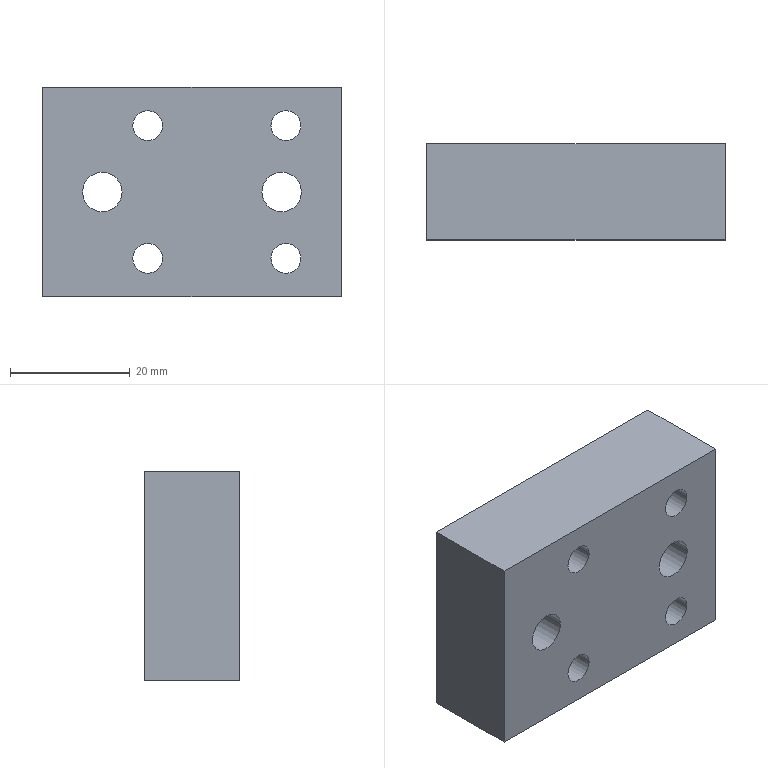Component | SolidWorks | QuickClampBackingPlate-1 | 1 solid | 24 faces | box 50 x 16 x 35 mm | volume 24821 mm3 | cylinder 16 | plane 8 | commonest cylinder face diameters 5 x8 11 x4 6.6 x4 | material 6061 Alloy
build123d program:
from build123d import *

# Parameters (mm, degrees)
SKETCH1_W                                          = 50
SKETCH1_H                                          = 35
BOSS_EXTRUDE1_DEPTH                                = 8
HOLE_SIZE_ACCORDING_TO_TYPE_1_OF_HEXAG_D           = 6.6
HOLE_SIZE_ACCORDING_TO_TYPE_1_OF_HEXAG_DEPTH       = 20
HOLE_SIZE_ACCORDING_TO_TYPE_1_OF_HEXAG_CBORE_D     = 11
HOLE_SIZE_ACCORDING_TO_TYPE_1_OF_HEXAG_CBORE_DEPTH = 6.8
HOLE_SIZE_ACCORDING_TO_TYPE_1_OF_HEXAG_TIP         = 1.983
M6_TAPPED_HOLE1_D                                  = 5
M6_TAPPED_HOLE1_DEPTH                              = 21
M6_TAPPED_HOLE1_TIP                                = 1.502


with BuildPart() as part:
    # Sketch1 → Boss-Extrude1 (new, symmetric)
    with BuildSketch(Plane.XY):
        Rectangle(SKETCH1_W, SKETCH1_H)
    extrude(amount=BOSS_EXTRUDE1_DEPTH, both=True)

    # Hole Size _according to_ Type 1 of Hexag
    with Locations(Plane(origin=(0, 0, -8), x_dir=(1, 0, 0), z_dir=(0, 0, -1))):
        with Locations((-15, 0), (15, 0)):
            CounterBoreHole(HOLE_SIZE_ACCORDING_TO_TYPE_1_OF_HEXAG_D / 2, HOLE_SIZE_ACCORDING_TO_TYPE_1_OF_HEXAG_CBORE_D / 2, HOLE_SIZE_ACCORDING_TO_TYPE_1_OF_HEXAG_CBORE_DEPTH, depth=HOLE_SIZE_ACCORDING_TO_TYPE_1_OF_HEXAG_DEPTH)
            with Locations((0, 0, -(HOLE_SIZE_ACCORDING_TO_TYPE_1_OF_HEXAG_DEPTH + HOLE_SIZE_ACCORDING_TO_TYPE_1_OF_HEXAG_TIP / 2))):  # 118° drill point
                Cone(0, HOLE_SIZE_ACCORDING_TO_TYPE_1_OF_HEXAG_D / 2, HOLE_SIZE_ACCORDING_TO_TYPE_1_OF_HEXAG_TIP, mode=Mode.SUBTRACT)

    # M6 Tapped Hole1
    with Locations(Plane(origin=(0, 0, -8), x_dir=(-1, 0, 0), z_dir=(0, 0, -1))):
        with Locations((-15.7, 11.1), (7.4, 11.1), (-15.7, -11.1), (7.4, -11.1)):
            Hole(M6_TAPPED_HOLE1_D / 2, depth=M6_TAPPED_HOLE1_DEPTH)
            with Locations((0, 0, -(M6_TAPPED_HOLE1_DEPTH + M6_TAPPED_HOLE1_TIP / 2))):  # 118° drill point
                Cone(0, M6_TAPPED_HOLE1_D / 2, M6_TAPPED_HOLE1_TIP, mode=Mode.SUBTRACT)


solid = part.part

# Placed as in the assembly
solid = solid.moved(Location((36.028, 36.101, 117.932), (90, 0, 0)))
STEP:
#1=COLOUR_RGB('',0.7922,0.8196,0.9333);
#2=FILL_AREA_STYLE_COLOUR('',#1);
#3=FILL_AREA_STYLE('',(#2));
#4=SURFACE_STYLE_FILL_AREA(#3);
#5=SURFACE_SIDE_STYLE('',(#4));
#6=SURFACE_STYLE_USAGE(.BOTH.,#5);
#7=PRESENTATION_STYLE_ASSIGNMENT((#6));
#8=CARTESIAN_POINT('',(2.135,1.106,5.08));
#9=VERTEX_POINT('',#8);
#10=CARTESIAN_POINT('',(1.938,1.106,5.08));
#11=VERTEX_POINT('',#10);
#12=CARTESIAN_POINT('',(2.037,1.106,5.08));
#13=DIRECTION('',(0.,1.,0.));
#14=DIRECTION('',(-1.,0.,0.));
#15=AXIS2_PLACEMENT_3D('',#12,#13,#14);
#16=CIRCLE('',#15,0.09843);
#17=EDGE_CURVE('',#9,#11,#16,.T.);
#18=ORIENTED_EDGE('',*,*,#17,.F.);
#19=CARTESIAN_POINT('',(2.135,1.736,5.08));
#20=VERTEX_POINT('',#19);
#21=CARTESIAN_POINT('',(2.135,1.736,5.08));
#22=DIRECTION('',(0.,1.,0.));
#23=VECTOR('',#22,39.37);
#24=LINE('',#21,#23);
#25=EDGE_CURVE('',#9,#20,#24,.T.);
#26=ORIENTED_EDGE('',*,*,#25,.T.);
#27=CARTESIAN_POINT('',(1.938,1.736,5.08));
#28=VERTEX_POINT('',#27);
#29=CARTESIAN_POINT('',(2.037,1.736,5.08));
#30=DIRECTION('',(0.,1.,0.));
#31=DIRECTION('',(-1.,0.,0.));
#32=AXIS2_PLACEMENT_3D('',#29,#30,#31);
#33=CIRCLE('',#32,0.09843);
#34=EDGE_CURVE('',#20,#28,#33,.T.);
#35=ORIENTED_EDGE('',*,*,#34,.T.);
#36=CARTESIAN_POINT('',(1.938,1.736,5.08));
#37=DIRECTION('',(0.,1.,0.));
#38=VECTOR('',#37,39.37);
#39=LINE('',#36,#38);
#40=EDGE_CURVE('',#11,#28,#39,.T.);
#41=ORIENTED_EDGE('',*,*,#40,.F.);
#42=EDGE_LOOP('',(#18,#26,#35,#41));
#43=FACE_OUTER_BOUND('',#42,.T.);
#44=CARTESIAN_POINT('',(2.037,1.736,5.08));
#45=DIRECTION('',(0.,1.,0.));
#46=DIRECTION('',(-1.,0.,0.));
#47=AXIS2_PLACEMENT_3D('',#44,#45,#46);
#48=CYLINDRICAL_SURFACE('',#47,0.09843);
#49=ADVANCED_FACE('',(#43),#48,.F.);
#50=CARTESIAN_POINT('',(1.226,1.106,5.08));
#51=VERTEX_POINT('',#50);
#52=CARTESIAN_POINT('',(1.029,1.106,5.08));
#53=VERTEX_POINT('',#52);
#54=CARTESIAN_POINT('',(1.127,1.106,5.08));
#55=DIRECTION('',(0.,1.,0.));
#56=DIRECTION('',(-1.,0.,0.));
#57=AXIS2_PLACEMENT_3D('',#54,#55,#56);
#58=CIRCLE('',#57,0.09843);
#59=EDGE_CURVE('',#51,#53,#58,.T.);
#60=ORIENTED_EDGE('',*,*,#59,.F.);
#61=CARTESIAN_POINT('',(1.226,1.736,5.08));
#62=VERTEX_POINT('',#61);
#63=CARTESIAN_POINT('',(1.226,1.736,5.08));
#64=DIRECTION('',(0.,1.,0.));
#65=VECTOR('',#64,39.37);
#66=LINE('',#63,#65);
#67=EDGE_CURVE('',#51,#62,#66,.T.);
#68=ORIENTED_EDGE('',*,*,#67,.T.);
#69=CARTESIAN_POINT('',(1.029,1.736,5.08));
#70=VERTEX_POINT('',#69);
#71=CARTESIAN_POINT('',(1.127,1.736,5.08));
#72=DIRECTION('',(0.,1.,0.));
#73=DIRECTION('',(-1.,0.,0.));
#74=AXIS2_PLACEMENT_3D('',#71,#72,#73);
#75=CIRCLE('',#74,0.09843);
#76=EDGE_CURVE('',#62,#70,#75,.T.);
#77=ORIENTED_EDGE('',*,*,#76,.T.);
#78=CARTESIAN_POINT('',(1.029,1.736,5.08));
#79=DIRECTION('',(0.,1.,0.));
#80=VECTOR('',#79,39.37);
#81=LINE('',#78,#80);
#82=EDGE_CURVE('',#53,#70,#81,.T.);
#83=ORIENTED_EDGE('',*,*,#82,.F.);
#84=EDGE_LOOP('',(#60,#68,#77,#83));
#85=FACE_OUTER_BOUND('',#84,.T.);
#86=CARTESIAN_POINT('',(1.127,1.736,5.08));
#87=DIRECTION('',(0.,1.,0.));
#88=DIRECTION('',(-1.,0.,0.));
#89=AXIS2_PLACEMENT_3D('',#86,#87,#88);
#90=CYLINDRICAL_SURFACE('',#89,0.09843);
#91=ADVANCED_FACE('',(#85),#90,.F.);
#92=CARTESIAN_POINT('',(2.135,1.106,4.206));
#93=VERTEX_POINT('',#92);
#94=CARTESIAN_POINT('',(1.938,1.106,4.206));
#95=VERTEX_POINT('',#94);
#96=CARTESIAN_POINT('',(2.037,1.106,4.206));
#97=DIRECTION('',(0.,1.,0.));
#98=DIRECTION('',(-1.,0.,0.));
#99=AXIS2_PLACEMENT_3D('',#96,#97,#98);
#100=CIRCLE('',#99,0.09843);
#101=EDGE_CURVE('',#93,#95,#100,.T.);
#102=ORIENTED_EDGE('',*,*,#101,.F.);
#103=CARTESIAN_POINT('',(2.135,1.736,4.206));
#104=VERTEX_POINT('',#103);
#105=CARTESIAN_POINT('',(2.135,1.736,4.206));
#106=DIRECTION('',(0.,1.,0.));
#107=VECTOR('',#106,39.37);
#108=LINE('',#105,#107);
#109=EDGE_CURVE('',#93,#104,#108,.T.);
#110=ORIENTED_EDGE('',*,*,#109,.T.);
#111=CARTESIAN_POINT('',(1.938,1.736,4.206));
#112=VERTEX_POINT('',#111);
#113=CARTESIAN_POINT('',(2.037,1.736,4.206));
#114=DIRECTION('',(0.,1.,0.));
#115=DIRECTION('',(-1.,0.,0.));
#116=AXIS2_PLACEMENT_3D('',#113,#114,#115);
#117=CIRCLE('',#116,0.09843);
#118=EDGE_CURVE('',#104,#112,#117,.T.);
#119=ORIENTED_EDGE('',*,*,#118,.T.);
#120=CARTESIAN_POINT('',(1.938,1.736,4.206));
#121=DIRECTION('',(0.,1.,0.));
#122=VECTOR('',#121,39.37);
#123=LINE('',#120,#122);
#124=EDGE_CURVE('',#95,#112,#123,.T.);
#125=ORIENTED_EDGE('',*,*,#124,.F.);
#126=EDGE_LOOP('',(#102,#110,#119,#125));
#127=FACE_OUTER_BOUND('',#126,.T.);
#128=CARTESIAN_POINT('',(2.037,1.736,4.206));
#129=DIRECTION('',(0.,1.,0.));
#130=DIRECTION('',(-1.,0.,0.));
#131=AXIS2_PLACEMENT_3D('',#128,#129,#130);
#132=CYLINDRICAL_SURFACE('',#131,0.09843);
#133=ADVANCED_FACE('',(#127),#132,.F.);
#134=CARTESIAN_POINT('',(1.226,1.106,4.206));
#135=VERTEX_POINT('',#134);
#136=CARTESIAN_POINT('',(1.029,1.106,4.206));
#137=VERTEX_POINT('',#136);
#138=CARTESIAN_POINT('',(1.127,1.106,4.206));
#139=DIRECTION('',(0.,1.,0.));
#140=DIRECTION('',(-1.,0.,0.));
#141=AXIS2_PLACEMENT_3D('',#138,#139,#140);
#142=CIRCLE('',#141,0.09843);
#143=EDGE_CURVE('',#135,#137,#142,.T.);
#144=ORIENTED_EDGE('',*,*,#143,.F.);
#145=CARTESIAN_POINT('',(1.226,1.736,4.206));
#146=VERTEX_POINT('',#145);
#147=CARTESIAN_POINT('',(1.226,1.736,4.206));
#148=DIRECTION('',(0.,1.,0.));
#149=VECTOR('',#148,39.37);
#150=LINE('',#147,#149);
#151=EDGE_CURVE('',#135,#146,#150,.T.);
#152=ORIENTED_EDGE('',*,*,#151,.T.);
#153=CARTESIAN_POINT('',(1.029,1.736,4.206));
#154=VERTEX_POINT('',#153);
#155=CARTESIAN_POINT('',(1.127,1.736,4.206));
#156=DIRECTION('',(0.,1.,0.));
#157=DIRECTION('',(-1.,0.,0.));
#158=AXIS2_PLACEMENT_3D('',#155,#156,#157);
#159=CIRCLE('',#158,0.09843);
#160=EDGE_CURVE('',#146,#154,#159,.T.);
#161=ORIENTED_EDGE('',*,*,#160,.T.);
#162=CARTESIAN_POINT('',(1.029,1.736,4.206));
#163=DIRECTION('',(0.,1.,0.));
#164=VECTOR('',#163,39.37);
#165=LINE('',#162,#164);
#166=EDGE_CURVE('',#137,#154,#165,.T.);
#167=ORIENTED_EDGE('',*,*,#166,.F.);
#168=EDGE_LOOP('',(#144,#152,#161,#167));
#169=FACE_OUTER_BOUND('',#168,.T.);
#170=CARTESIAN_POINT('',(1.127,1.736,4.206));
#171=DIRECTION('',(0.,1.,0.));
#172=DIRECTION('',(-1.,0.,0.));
#173=AXIS2_PLACEMENT_3D('',#170,#171,#172);
#174=CYLINDRICAL_SURFACE('',#173,0.09843);
#175=ADVANCED_FACE('',(#169),#174,.F.);
#176=CARTESIAN_POINT('',(1.044,1.469,4.643));
#177=VERTEX_POINT('',#176);
#178=CARTESIAN_POINT('',(0.6113,1.469,4.643));
#179=VERTEX_POINT('',#178);
#180=CARTESIAN_POINT('',(0.8279,1.469,4.643));
#181=DIRECTION('',(0.,1.,0.));
#182=DIRECTION('',(-1.,0.,0.));
#183=AXIS2_PLACEMENT_3D('',#180,#181,#182);
#184=CIRCLE('',#183,0.2165);
#185=EDGE_CURVE('',#177,#179,#184,.T.);
#186=ORIENTED_EDGE('',*,*,#185,.F.);
#187=CARTESIAN_POINT('',(1.044,1.736,4.643));
#188=VERTEX_POINT('',#187);
#189=CARTESIAN_POINT('',(1.044,1.736,4.643));
#190=DIRECTION('',(0.,1.,0.));
#191=VECTOR('',#190,39.37);
#192=LINE('',#189,#191);
#193=EDGE_CURVE('',#177,#188,#192,.T.);
#194=ORIENTED_EDGE('',*,*,#193,.T.);
#195=CARTESIAN_POINT('',(0.6113,1.736,4.643));
#196=VERTEX_POINT('',#195);
#197=CARTESIAN_POINT('',(0.8279,1.736,4.643));
#198=DIRECTION('',(0.,1.,0.));
#199=DIRECTION('',(-1.,0.,0.));
#200=AXIS2_PLACEMENT_3D('',#197,#198,#199);
#201=CIRCLE('',#200,0.2165);
#202=EDGE_CURVE('',#188,#196,#201,.T.);
#203=ORIENTED_EDGE('',*,*,#202,.T.);
#204=CARTESIAN_POINT('',(0.6113,1.736,4.643));
#205=DIRECTION('',(0.,1.,0.));
#206=VECTOR('',#205,39.37);
#207=LINE('',#204,#206);
#208=EDGE_CURVE('',#179,#196,#207,.T.);
#209=ORIENTED_EDGE('',*,*,#208,.F.);
#210=EDGE_LOOP('',(#186,#194,#203,#209));
#211=FACE_OUTER_BOUND('',#210,.T.);
#212=CARTESIAN_POINT('',(0.8279,1.736,4.643));
#213=DIRECTION('',(0.,1.,0.));
#214=DIRECTION('',(-1.,0.,0.));
#215=AXIS2_PLACEMENT_3D('',#212,#213,#214);
#216=CYLINDRICAL_SURFACE('',#215,0.2165);
#217=ADVANCED_FACE('',(#211),#216,.F.);
#218=CARTESIAN_POINT('',(0.9578,1.106,4.643));
#219=VERTEX_POINT('',#218);
#220=CARTESIAN_POINT('',(0.698,1.106,4.643));
#221=VERTEX_POINT('',#220);
#222=CARTESIAN_POINT('',(0.8279,1.106,4.643));
#223=DIRECTION('',(0.,1.,0.));
#224=DIRECTION('',(-1.,0.,0.));
#225=AXIS2_PLACEMENT_3D('',#222,#223,#224);
#226=CIRCLE('',#225,0.1299);
#227=EDGE_CURVE('',#219,#221,#226,.T.);
#228=ORIENTED_EDGE('',*,*,#227,.F.);
#229=CARTESIAN_POINT('',(0.9578,1.469,4.643));
#230=VERTEX_POINT('',#229);
#231=CARTESIAN_POINT('',(0.9578,1.736,4.643));
#232=DIRECTION('',(0.,1.,0.));
#233=VECTOR('',#232,39.37);
#234=LINE('',#231,#233);
#235=EDGE_CURVE('',#219,#230,#234,.T.);
#236=ORIENTED_EDGE('',*,*,#235,.T.);
#237=CARTESIAN_POINT('',(0.698,1.469,4.643));
#238=VERTEX_POINT('',#237);
#239=CARTESIAN_POINT('',(0.8279,1.469,4.643));
#240=DIRECTION('',(0.,1.,0.));
#241=DIRECTION('',(-1.,0.,0.));
#242=AXIS2_PLACEMENT_3D('',#239,#240,#241);
#243=CIRCLE('',#242,0.1299);
#244=EDGE_CURVE('',#230,#238,#243,.T.);
#245=ORIENTED_EDGE('',*,*,#244,.T.);
#246=CARTESIAN_POINT('',(0.698,1.736,4.643));
#247=DIRECTION('',(0.,1.,0.));
#248=VECTOR('',#247,39.37);
#249=LINE('',#246,#248);
#250=EDGE_CURVE('',#221,#238,#249,.T.);
#251=ORIENTED_EDGE('',*,*,#250,.F.);
#252=EDGE_LOOP('',(#228,#236,#245,#251));
#253=FACE_OUTER_BOUND('',#252,.T.);
#254=CARTESIAN_POINT('',(0.8279,1.736,4.643));
#255=DIRECTION('',(0.,1.,0.));
#256=DIRECTION('',(-1.,0.,0.));
#257=AXIS2_PLACEMENT_3D('',#254,#255,#256);
#258=CYLINDRICAL_SURFACE('',#257,0.1299);
#259=ADVANCED_FACE('',(#253),#258,.F.);
#260=CARTESIAN_POINT('',(2.226,1.469,4.643));
#261=VERTEX_POINT('',#260);
#262=CARTESIAN_POINT('',(1.792,1.469,4.643));
#263=VERTEX_POINT('',#262);
#264=CARTESIAN_POINT('',(2.009,1.469,4.643));
#265=DIRECTION('',(0.,1.,0.));
#266=DIRECTION('',(-1.,0.,0.));
#267=AXIS2_PLACEMENT_3D('',#264,#265,#266);
#268=CIRCLE('',#267,0.2165);
#269=EDGE_CURVE('',#261,#263,#268,.T.);
#270=ORIENTED_EDGE('',*,*,#269,.F.);
#271=CARTESIAN_POINT('',(2.226,1.736,4.643));
#272=VERTEX_POINT('',#271);
#273=CARTESIAN_POINT('',(2.226,1.736,4.643));
#274=DIRECTION('',(0.,1.,0.));
#275=VECTOR('',#274,39.37);
#276=LINE('',#273,#275);
#277=EDGE_CURVE('',#261,#272,#276,.T.);
#278=ORIENTED_EDGE('',*,*,#277,.T.);
#279=CARTESIAN_POINT('',(1.792,1.736,4.643));
#280=VERTEX_POINT('',#279);
#281=CARTESIAN_POINT('',(2.009,1.736,4.643));
#282=DIRECTION('',(0.,1.,0.));
#283=DIRECTION('',(-1.,0.,0.));
#284=AXIS2_PLACEMENT_3D('',#281,#282,#283);
#285=CIRCLE('',#284,0.2165);
#286=EDGE_CURVE('',#272,#280,#285,.T.);
#287=ORIENTED_EDGE('',*,*,#286,.T.);
#288=CARTESIAN_POINT('',(1.792,1.736,4.643));
#289=DIRECTION('',(0.,1.,0.));
#290=VECTOR('',#289,39.37);
#291=LINE('',#288,#290);
#292=EDGE_CURVE('',#263,#280,#291,.T.);
#293=ORIENTED_EDGE('',*,*,#292,.F.);
#294=EDGE_LOOP('',(#270,#278,#287,#293));
#295=FACE_OUTER_BOUND('',#294,.T.);
#296=CARTESIAN_POINT('',(2.009,1.736,4.643));
#297=DIRECTION('',(0.,1.,0.));
#298=DIRECTION('',(-1.,0.,0.));
#299=AXIS2_PLACEMENT_3D('',#296,#297,#298);
#300=CYLINDRICAL_SURFACE('',#299,0.2165);
#301=ADVANCED_FACE('',(#295),#300,.F.);
#302=CARTESIAN_POINT('',(2.139,1.106,4.643));
#303=VERTEX_POINT('',#302);
#304=CARTESIAN_POINT('',(1.879,1.106,4.643));
#305=VERTEX_POINT('',#304);
#306=CARTESIAN_POINT('',(2.009,1.106,4.643));
#307=DIRECTION('',(0.,1.,0.));
#308=DIRECTION('',(-1.,0.,0.));
#309=AXIS2_PLACEMENT_3D('',#306,#307,#308);
#310=CIRCLE('',#309,0.1299);
#311=EDGE_CURVE('',#303,#305,#310,.T.);
#312=ORIENTED_EDGE('',*,*,#311,.F.);
#313=CARTESIAN_POINT('',(2.139,1.469,4.643));
#314=VERTEX_POINT('',#313);
#315=CARTESIAN_POINT('',(2.139,1.736,4.643));
#316=DIRECTION('',(0.,1.,0.));
#317=VECTOR('',#316,39.37);
#318=LINE('',#315,#317);
#319=EDGE_CURVE('',#303,#314,#318,.T.);
#320=ORIENTED_EDGE('',*,*,#319,.T.);
#321=CARTESIAN_POINT('',(1.879,1.469,4.643));
#322=VERTEX_POINT('',#321);
#323=CARTESIAN_POINT('',(2.009,1.469,4.643));
#324=DIRECTION('',(0.,1.,0.));
#325=DIRECTION('',(-1.,0.,0.));
#326=AXIS2_PLACEMENT_3D('',#323,#324,#325);
#327=CIRCLE('',#326,0.1299);
#328=EDGE_CURVE('',#314,#322,#327,.T.);
#329=ORIENTED_EDGE('',*,*,#328,.T.);
#330=CARTESIAN_POINT('',(1.879,1.736,4.643));
#331=DIRECTION('',(0.,1.,0.));
#332=VECTOR('',#331,39.37);
#333=LINE('',#330,#332);
#334=EDGE_CURVE('',#305,#322,#333,.T.);
#335=ORIENTED_EDGE('',*,*,#334,.F.);
#336=EDGE_LOOP('',(#312,#320,#329,#335));
#337=FACE_OUTER_BOUND('',#336,.T.);
#338=CARTESIAN_POINT('',(2.009,1.736,4.643));
#339=DIRECTION('',(0.,1.,0.));
#340=DIRECTION('',(-1.,0.,0.));
#341=AXIS2_PLACEMENT_3D('',#338,#339,#340);
#342=CYLINDRICAL_SURFACE('',#341,0.1299);
#343=ADVANCED_FACE('',(#337),#342,.F.);
#344=CARTESIAN_POINT('',(0.4342,1.736,5.332));
#345=VERTEX_POINT('',#344);
#346=CARTESIAN_POINT('',(0.4342,1.736,3.954));
#347=VERTEX_POINT('',#346);
#348=CARTESIAN_POINT('',(0.4342,1.736,5.332));
#349=DIRECTION('',(0.,0.,-1.));
#350=VECTOR('',#349,39.37);
#351=LINE('',#348,#350);
#352=EDGE_CURVE('',#345,#347,#351,.T.);
#353=ORIENTED_EDGE('',*,*,#352,.T.);
#354=CARTESIAN_POINT('',(0.4342,1.106,3.954));
#355=VERTEX_POINT('',#354);
#356=CARTESIAN_POINT('',(0.4342,1.106,3.954));
#357=DIRECTION('',(0.,1.,0.));
#358=VECTOR('',#357,39.37);
#359=LINE('',#356,#358);
#360=EDGE_CURVE('',#355,#347,#359,.T.);
#361=ORIENTED_EDGE('',*,*,#360,.F.);
#362=CARTESIAN_POINT('',(0.4342,1.106,5.332));
#363=VERTEX_POINT('',#362);
#364=CARTESIAN_POINT('',(0.4342,1.106,5.332));
#365=DIRECTION('',(0.,0.,-1.));
#366=VECTOR('',#365,39.37);
#367=LINE('',#364,#366);
#368=EDGE_CURVE('',#363,#355,#367,.T.);
#369=ORIENTED_EDGE('',*,*,#368,.F.);
#370=CARTESIAN_POINT('',(0.4342,1.106,5.332));
#371=DIRECTION('',(0.,1.,0.));
#372=VECTOR('',#371,39.37);
#373=LINE('',#370,#372);
#374=EDGE_CURVE('',#363,#345,#373,.T.);
#375=ORIENTED_EDGE('',*,*,#374,.T.);
#376=EDGE_LOOP('',(#353,#361,#369,#375));
#377=FACE_OUTER_BOUND('',#376,.T.);
#378=CARTESIAN_POINT('',(0.4342,1.106,5.332));
#379=DIRECTION('',(1.,0.,0.));
#380=DIRECTION('',(-0.,0.,1.));
#381=AXIS2_PLACEMENT_3D('',#378,#379,#380);
#382=PLANE('',#381);
#383=ADVANCED_FACE('',(#377),#382,.F.);
#384=CARTESIAN_POINT('',(2.403,1.736,3.954));
#385=VERTEX_POINT('',#384);
#386=CARTESIAN_POINT('',(2.403,1.736,3.954));
#387=DIRECTION('',(1.,0.,0.));
#388=VECTOR('',#387,39.37);
#389=LINE('',#386,#388);
#390=EDGE_CURVE('',#347,#385,#389,.T.);
#391=ORIENTED_EDGE('',*,*,#390,.T.);
#392=CARTESIAN_POINT('',(2.403,1.106,3.954));
#393=VERTEX_POINT('',#392);
#394=CARTESIAN_POINT('',(2.403,1.106,3.954));
#395=DIRECTION('',(0.,1.,0.));
#396=VECTOR('',#395,39.37);
#397=LINE('',#394,#396);
#398=EDGE_CURVE('',#393,#385,#397,.T.);
#399=ORIENTED_EDGE('',*,*,#398,.F.);
#400=CARTESIAN_POINT('',(2.403,1.106,3.954));
#401=DIRECTION('',(1.,0.,0.));
#402=VECTOR('',#401,39.37);
#403=LINE('',#400,#402);
#404=EDGE_CURVE('',#355,#393,#403,.T.);
#405=ORIENTED_EDGE('',*,*,#404,.F.);
#406=ORIENTED_EDGE('',*,*,#360,.T.);
#407=EDGE_LOOP('',(#391,#399,#405,#406));
#408=FACE_OUTER_BOUND('',#407,.T.);
#409=CARTESIAN_POINT('',(2.403,1.106,3.954));
#410=DIRECTION('',(-0.,0.,1.));
#411=DIRECTION('',(-1.,0.,-0.));
#412=AXIS2_PLACEMENT_3D('',#409,#410,#411);
#413=PLANE('',#412);
#414=ADVANCED_FACE('',(#408),#413,.F.);
#415=CARTESIAN_POINT('',(2.403,1.736,5.332));
#416=VERTEX_POINT('',#415);
#417=CARTESIAN_POINT('',(2.403,1.736,5.332));
#418=DIRECTION('',(-0.,0.,1.));
#419=VECTOR('',#418,39.37);
#420=LINE('',#417,#419);
#421=EDGE_CURVE('',#385,#416,#420,.T.);
#422=ORIENTED_EDGE('',*,*,#421,.T.);
#423=CARTESIAN_POINT('',(2.403,1.106,5.332));
#424=VERTEX_POINT('',#423);
#425=CARTESIAN_POINT('',(2.403,1.106,5.332));
#426=DIRECTION('',(0.,1.,0.));
#427=VECTOR('',#426,39.37);
#428=LINE('',#425,#427);
#429=EDGE_CURVE('',#424,#416,#428,.T.);
#430=ORIENTED_EDGE('',*,*,#429,.F.);
#431=CARTESIAN_POINT('',(2.403,1.106,5.332));
#432=DIRECTION('',(-0.,0.,1.));
#433=VECTOR('',#432,39.37);
#434=LINE('',#431,#433);
#435=EDGE_CURVE('',#393,#424,#434,.T.);
#436=ORIENTED_EDGE('',*,*,#435,.F.);
#437=ORIENTED_EDGE('',*,*,#398,.T.);
#438=EDGE_LOOP('',(#422,#430,#436,#437));
#439=FACE_OUTER_BOUND('',#438,.T.);
#440=CARTESIAN_POINT('',(2.403,1.106,5.332));
#441=DIRECTION('',(-1.,0.,-0.));
#442=DIRECTION('',(0.,0.,-1.));
#443=AXIS2_PLACEMENT_3D('',#440,#441,#442);
#444=PLANE('',#443);
#445=ADVANCED_FACE('',(#439),#444,.F.);
#446=CARTESIAN_POINT('',(2.403,1.736,5.332));
#447=DIRECTION('',(-1.,0.,-0.));
#448=VECTOR('',#447,39.37);
#449=LINE('',#446,#448);
#450=EDGE_CURVE('',#416,#345,#449,.T.);
#451=ORIENTED_EDGE('',*,*,#450,.T.);
#452=ORIENTED_EDGE('',*,*,#374,.F.);
#453=CARTESIAN_POINT('',(2.403,1.106,5.332));
#454=DIRECTION('',(-1.,0.,-0.));
#455=VECTOR('',#454,39.37);
#456=LINE('',#453,#455);
#457=EDGE_CURVE('',#424,#363,#456,.T.);
#458=ORIENTED_EDGE('',*,*,#457,.F.);
#459=ORIENTED_EDGE('',*,*,#429,.T.);
#460=EDGE_LOOP('',(#451,#452,#458,#459));
#461=FACE_OUTER_BOUND('',#460,.T.);
#462=CARTESIAN_POINT('',(2.403,1.106,5.332));
#463=DIRECTION('',(0.,0.,-1.));
#464=DIRECTION('',(1.,0.,0.));
#465=AXIS2_PLACEMENT_3D('',#462,#463,#464);
#466=PLANE('',#465);
#467=ADVANCED_FACE('',(#461),#466,.F.);
#468=CARTESIAN_POINT('',(2.037,1.106,5.08));
#469=DIRECTION('',(0.,1.,0.));
#470=DIRECTION('',(-1.,0.,0.));
#471=AXIS2_PLACEMENT_3D('',#468,#469,#470);
#472=CIRCLE('',#471,0.09843);
#473=EDGE_CURVE('',#11,#9,#472,.T.);
#474=ORIENTED_EDGE('',*,*,#473,.T.);
#475=ORIENTED_EDGE('',*,*,#17,.T.);
#476=EDGE_LOOP('',(#474,#475));
#477=FACE_BOUND('',#476,.T.);
#478=CARTESIAN_POINT('',(1.127,1.106,5.08));
#479=DIRECTION('',(0.,1.,0.));
#480=DIRECTION('',(-1.,0.,0.));
#481=AXIS2_PLACEMENT_3D('',#478,#479,#480);
#482=CIRCLE('',#481,0.09843);
#483=EDGE_CURVE('',#53,#51,#482,.T.);
#484=ORIENTED_EDGE('',*,*,#483,.T.);
#485=ORIENTED_EDGE('',*,*,#59,.T.);
#486=EDGE_LOOP('',(#484,#485));
#487=FACE_BOUND('',#486,.T.);
#488=CARTESIAN_POINT('',(2.037,1.106,4.206));
#489=DIRECTION('',(0.,1.,0.));
#490=DIRECTION('',(-1.,0.,0.));
#491=AXIS2_PLACEMENT_3D('',#488,#489,#490);
#492=CIRCLE('',#491,0.09843);
#493=EDGE_CURVE('',#95,#93,#492,.T.);
#494=ORIENTED_EDGE('',*,*,#493,.T.);
#495=ORIENTED_EDGE('',*,*,#101,.T.);
#496=EDGE_LOOP('',(#494,#495));
#497=FACE_BOUND('',#496,.T.);
#498=CARTESIAN_POINT('',(1.127,1.106,4.206));
#499=DIRECTION('',(0.,1.,0.));
#500=DIRECTION('',(-1.,0.,0.));
#501=AXIS2_PLACEMENT_3D('',#498,#499,#500);
#502=CIRCLE('',#501,0.09843);
#503=EDGE_CURVE('',#137,#135,#502,.T.);
#504=ORIENTED_EDGE('',*,*,#503,.T.);
#505=ORIENTED_EDGE('',*,*,#143,.T.);
#506=EDGE_LOOP('',(#504,#505));
#507=FACE_BOUND('',#506,.T.);
#508=CARTESIAN_POINT('',(0.8279,1.106,4.643));
#509=DIRECTION('',(0.,1.,0.));
#510=DIRECTION('',(-1.,0.,0.));
#511=AXIS2_PLACEMENT_3D('',#508,#509,#510);
#512=CIRCLE('',#511,0.1299);
#513=EDGE_CURVE('',#221,#219,#512,.T.);
#514=ORIENTED_EDGE('',*,*,#513,.T.);
#515=ORIENTED_EDGE('',*,*,#227,.T.);
#516=EDGE_LOOP('',(#514,#515));
#517=FACE_BOUND('',#516,.T.);
#518=CARTESIAN_POINT('',(2.009,1.106,4.643));
#519=DIRECTION('',(0.,1.,0.));
#520=DIRECTION('',(-1.,0.,0.));
#521=AXIS2_PLACEMENT_3D('',#518,#519,#520);
#522=CIRCLE('',#521,0.1299);
#523=EDGE_CURVE('',#305,#303,#522,.T.);
#524=ORIENTED_EDGE('',*,*,#523,.T.);
#525=ORIENTED_EDGE('',*,*,#311,.T.);
#526=EDGE_LOOP('',(#524,#525));
#527=FACE_BOUND('',#526,.T.);
#528=ORIENTED_EDGE('',*,*,#368,.T.);
#529=ORIENTED_EDGE('',*,*,#404,.T.);
#530=ORIENTED_EDGE('',*,*,#435,.T.);
#531=ORIENTED_EDGE('',*,*,#457,.T.);
#532=EDGE_LOOP('',(#528,#529,#530,#531));
#533=FACE_OUTER_BOUND('',#532,.T.);
#534=CARTESIAN_POINT('',(1.418,1.106,4.643));
#535=DIRECTION('',(0.,1.,0.));
#536=DIRECTION('',(-1.,0.,0.));
#537=AXIS2_PLACEMENT_3D('',#534,#535,#536);
#538=PLANE('',#537);
#539=ADVANCED_FACE('',(#477,#487,#497,#507,#517,#527,#533),#538,.F.);
#540=CARTESIAN_POINT('',(2.037,1.736,5.08));
#541=DIRECTION('',(0.,1.,0.));
#542=DIRECTION('',(-1.,0.,0.));
#543=AXIS2_PLACEMENT_3D('',#540,#541,#542);
#544=CIRCLE('',#543,0.09843);
#545=EDGE_CURVE('',#28,#20,#544,.T.);
#546=ORIENTED_EDGE('',*,*,#545,.F.);
#547=ORIENTED_EDGE('',*,*,#34,.F.);
#548=EDGE_LOOP('',(#546,#547));
#549=FACE_BOUND('',#548,.T.);
#550=CARTESIAN_POINT('',(1.127,1.736,5.08));
#551=DIRECTION('',(0.,1.,0.));
#552=DIRECTION('',(-1.,0.,0.));
#553=AXIS2_PLACEMENT_3D('',#550,#551,#552);
#554=CIRCLE('',#553,0.09843);
#555=EDGE_CURVE('',#70,#62,#554,.T.);
#556=ORIENTED_EDGE('',*,*,#555,.F.);
#557=ORIENTED_EDGE('',*,*,#76,.F.);
#558=EDGE_LOOP('',(#556,#557));
#559=FACE_BOUND('',#558,.T.);
#560=CARTESIAN_POINT('',(2.037,1.736,4.206));
#561=DIRECTION('',(0.,1.,0.));
#562=DIRECTION('',(-1.,0.,0.));
#563=AXIS2_PLACEMENT_3D('',#560,#561,#562);
#564=CIRCLE('',#563,0.09843);
#565=EDGE_CURVE('',#112,#104,#564,.T.);
#566=ORIENTED_EDGE('',*,*,#565,.F.);
#567=ORIENTED_EDGE('',*,*,#118,.F.);
#568=EDGE_LOOP('',(#566,#567));
#569=FACE_BOUND('',#568,.T.);
#570=CARTESIAN_POINT('',(1.127,1.736,4.206));
#571=DIRECTION('',(0.,1.,0.));
#572=DIRECTION('',(-1.,0.,0.));
#573=AXIS2_PLACEMENT_3D('',#570,#571,#572);
#574=CIRCLE('',#573,0.09843);
#575=EDGE_CURVE('',#154,#146,#574,.T.);
#576=ORIENTED_EDGE('',*,*,#575,.F.);
#577=ORIENTED_EDGE('',*,*,#160,.F.);
#578=EDGE_LOOP('',(#576,#577));
#579=FACE_BOUND('',#578,.T.);
#580=CARTESIAN_POINT('',(0.8279,1.736,4.643));
#581=DIRECTION('',(0.,1.,0.));
#582=DIRECTION('',(-1.,0.,0.));
#583=AXIS2_PLACEMENT_3D('',#580,#581,#582);
#584=CIRCLE('',#583,0.2165);
#585=EDGE_CURVE('',#196,#188,#584,.T.);
#586=ORIENTED_EDGE('',*,*,#585,.F.);
#587=ORIENTED_EDGE('',*,*,#202,.F.);
#588=EDGE_LOOP('',(#586,#587));
#589=FACE_BOUND('',#588,.T.);
#590=CARTESIAN_POINT('',(2.009,1.736,4.643));
#591=DIRECTION('',(0.,1.,0.));
#592=DIRECTION('',(-1.,0.,0.));
#593=AXIS2_PLACEMENT_3D('',#590,#591,#592);
#594=CIRCLE('',#593,0.2165);
#595=EDGE_CURVE('',#280,#272,#594,.T.);
#596=ORIENTED_EDGE('',*,*,#595,.F.);
#597=ORIENTED_EDGE('',*,*,#286,.F.);
#598=EDGE_LOOP('',(#596,#597));
#599=FACE_BOUND('',#598,.T.);
#600=ORIENTED_EDGE('',*,*,#352,.F.);
#601=ORIENTED_EDGE('',*,*,#450,.F.);
#602=ORIENTED_EDGE('',*,*,#421,.F.);
#603=ORIENTED_EDGE('',*,*,#390,.F.);
#604=EDGE_LOOP('',(#600,#601,#602,#603));
#605=FACE_OUTER_BOUND('',#604,.T.);
#606=CARTESIAN_POINT('',(1.418,1.736,4.643));
#607=DIRECTION('',(0.,1.,0.));
#608=DIRECTION('',(-1.,0.,0.));
#609=AXIS2_PLACEMENT_3D('',#606,#607,#608);
#610=PLANE('',#609);
#611=ADVANCED_FACE('',(#549,#559,#569,#579,#589,#599,#605),#610,.T.);
#612=ORIENTED_EDGE('',*,*,#319,.F.);
#613=ORIENTED_EDGE('',*,*,#523,.F.);
#614=ORIENTED_EDGE('',*,*,#334,.T.);
#615=CARTESIAN_POINT('',(2.009,1.469,4.643));
#616=DIRECTION('',(0.,1.,0.));
#617=DIRECTION('',(-1.,0.,0.));
#618=AXIS2_PLACEMENT_3D('',#615,#616,#617);
#619=CIRCLE('',#618,0.1299);
#620=EDGE_CURVE('',#322,#314,#619,.T.);
#621=ORIENTED_EDGE('',*,*,#620,.T.);
#622=EDGE_LOOP('',(#612,#613,#614,#621));
#623=FACE_OUTER_BOUND('',#622,.T.);
#624=CARTESIAN_POINT('',(2.009,1.736,4.643));
#625=DIRECTION('',(0.,1.,0.));
#626=DIRECTION('',(-1.,0.,0.));
#627=AXIS2_PLACEMENT_3D('',#624,#625,#626);
#628=CYLINDRICAL_SURFACE('',#627,0.1299);
#629=ADVANCED_FACE('',(#623),#628,.F.);
#630=ORIENTED_EDGE('',*,*,#620,.F.);
#631=ORIENTED_EDGE('',*,*,#328,.F.);
#632=EDGE_LOOP('',(#630,#631));
#633=FACE_BOUND('',#632,.T.);
#634=CARTESIAN_POINT('',(2.009,1.469,4.643));
#635=DIRECTION('',(0.,1.,0.));
#636=DIRECTION('',(-1.,0.,0.));
#637=AXIS2_PLACEMENT_3D('',#634,#635,#636);
#638=CIRCLE('',#637,0.2165);
#639=EDGE_CURVE('',#263,#261,#638,.T.);
#640=ORIENTED_EDGE('',*,*,#639,.T.);
#641=ORIENTED_EDGE('',*,*,#269,.T.);
#642=EDGE_LOOP('',(#640,#641));
#643=FACE_OUTER_BOUND('',#642,.T.);
#644=CARTESIAN_POINT('',(2.139,1.469,4.643));
#645=DIRECTION('',(0.,-1.,0.));
#646=DIRECTION('',(1.,0.,0.));
#647=AXIS2_PLACEMENT_3D('',#644,#645,#646);
#648=PLANE('',#647);
#649=ADVANCED_FACE('',(#633,#643),#648,.F.);
#650=ORIENTED_EDGE('',*,*,#277,.F.);
#651=ORIENTED_EDGE('',*,*,#639,.F.);
#652=ORIENTED_EDGE('',*,*,#292,.T.);
#653=ORIENTED_EDGE('',*,*,#595,.T.);
#654=EDGE_LOOP('',(#650,#651,#652,#653));
#655=FACE_OUTER_BOUND('',#654,.T.);
#656=CARTESIAN_POINT('',(2.009,1.736,4.643));
#657=DIRECTION('',(0.,1.,0.));
#658=DIRECTION('',(-1.,0.,0.));
#659=AXIS2_PLACEMENT_3D('',#656,#657,#658);
#660=CYLINDRICAL_SURFACE('',#659,0.2165);
#661=ADVANCED_FACE('',(#655),#660,.F.);
#662=ORIENTED_EDGE('',*,*,#235,.F.);
#663=ORIENTED_EDGE('',*,*,#513,.F.);
#664=ORIENTED_EDGE('',*,*,#250,.T.);
#665=CARTESIAN_POINT('',(0.8279,1.469,4.643));
#666=DIRECTION('',(0.,1.,0.));
#667=DIRECTION('',(-1.,0.,0.));
#668=AXIS2_PLACEMENT_3D('',#665,#666,#667);
#669=CIRCLE('',#668,0.1299);
#670=EDGE_CURVE('',#238,#230,#669,.T.);
#671=ORIENTED_EDGE('',*,*,#670,.T.);
#672=EDGE_LOOP('',(#662,#663,#664,#671));
#673=FACE_OUTER_BOUND('',#672,.T.);
#674=CARTESIAN_POINT('',(0.8279,1.736,4.643));
#675=DIRECTION('',(0.,1.,0.));
#676=DIRECTION('',(-1.,0.,0.));
#677=AXIS2_PLACEMENT_3D('',#674,#675,#676);
#678=CYLINDRICAL_SURFACE('',#677,0.1299);
#679=ADVANCED_FACE('',(#673),#678,.F.);
#680=ORIENTED_EDGE('',*,*,#670,.F.);
#681=ORIENTED_EDGE('',*,*,#244,.F.);
#682=EDGE_LOOP('',(#680,#681));
#683=FACE_BOUND('',#682,.T.);
#684=CARTESIAN_POINT('',(0.8279,1.469,4.643));
#685=DIRECTION('',(0.,1.,0.));
#686=DIRECTION('',(-1.,0.,0.));
#687=AXIS2_PLACEMENT_3D('',#684,#685,#686);
#688=CIRCLE('',#687,0.2165);
#689=EDGE_CURVE('',#179,#177,#688,.T.);
#690=ORIENTED_EDGE('',*,*,#689,.T.);
#691=ORIENTED_EDGE('',*,*,#185,.T.);
#692=EDGE_LOOP('',(#690,#691));
#693=FACE_OUTER_BOUND('',#692,.T.);
#694=CARTESIAN_POINT('',(0.9578,1.469,4.643));
#695=DIRECTION('',(0.,-1.,0.));
#696=DIRECTION('',(1.,0.,0.));
#697=AXIS2_PLACEMENT_3D('',#694,#695,#696);
#698=PLANE('',#697);
#699=ADVANCED_FACE('',(#683,#693),#698,.F.);
#700=ORIENTED_EDGE('',*,*,#193,.F.);
#701=ORIENTED_EDGE('',*,*,#689,.F.);
#702=ORIENTED_EDGE('',*,*,#208,.T.);
#703=ORIENTED_EDGE('',*,*,#585,.T.);
#704=EDGE_LOOP('',(#700,#701,#702,#703));
#705=FACE_OUTER_BOUND('',#704,.T.);
#706=CARTESIAN_POINT('',(0.8279,1.736,4.643));
#707=DIRECTION('',(0.,1.,0.));
#708=DIRECTION('',(-1.,0.,0.));
#709=AXIS2_PLACEMENT_3D('',#706,#707,#708);
#710=CYLINDRICAL_SURFACE('',#709,0.2165);
#711=ADVANCED_FACE('',(#705),#710,.F.);
#712=ORIENTED_EDGE('',*,*,#151,.F.);
#713=ORIENTED_EDGE('',*,*,#503,.F.);
#714=ORIENTED_EDGE('',*,*,#166,.T.);
#715=ORIENTED_EDGE('',*,*,#575,.T.);
#716=EDGE_LOOP('',(#712,#713,#714,#715));
#717=FACE_OUTER_BOUND('',#716,.T.);
#718=CARTESIAN_POINT('',(1.127,1.736,4.206));
#719=DIRECTION('',(0.,1.,0.));
#720=DIRECTION('',(-1.,0.,0.));
#721=AXIS2_PLACEMENT_3D('',#718,#719,#720);
#722=CYLINDRICAL_SURFACE('',#721,0.09843);
#723=ADVANCED_FACE('',(#717),#722,.F.);
#724=ORIENTED_EDGE('',*,*,#109,.F.);
#725=ORIENTED_EDGE('',*,*,#493,.F.);
#726=ORIENTED_EDGE('',*,*,#124,.T.);
#727=ORIENTED_EDGE('',*,*,#565,.T.);
#728=EDGE_LOOP('',(#724,#725,#726,#727));
#729=FACE_OUTER_BOUND('',#728,.T.);
#730=CARTESIAN_POINT('',(2.037,1.736,4.206));
#731=DIRECTION('',(0.,1.,0.));
#732=DIRECTION('',(-1.,0.,0.));
#733=AXIS2_PLACEMENT_3D('',#730,#731,#732);
#734=CYLINDRICAL_SURFACE('',#733,0.09843);
#735=ADVANCED_FACE('',(#729),#734,.F.);
#736=ORIENTED_EDGE('',*,*,#67,.F.);
#737=ORIENTED_EDGE('',*,*,#483,.F.);
#738=ORIENTED_EDGE('',*,*,#82,.T.);
#739=ORIENTED_EDGE('',*,*,#555,.T.);
#740=EDGE_LOOP('',(#736,#737,#738,#739));
#741=FACE_OUTER_BOUND('',#740,.T.);
#742=CARTESIAN_POINT('',(1.127,1.736,5.08));
#743=DIRECTION('',(0.,1.,0.));
#744=DIRECTION('',(-1.,0.,0.));
#745=AXIS2_PLACEMENT_3D('',#742,#743,#744);
#746=CYLINDRICAL_SURFACE('',#745,0.09843);
#747=ADVANCED_FACE('',(#741),#746,.F.);
#748=ORIENTED_EDGE('',*,*,#25,.F.);
#749=ORIENTED_EDGE('',*,*,#473,.F.);
#750=ORIENTED_EDGE('',*,*,#40,.T.);
#751=ORIENTED_EDGE('',*,*,#545,.T.);
#752=EDGE_LOOP('',(#748,#749,#750,#751));
#753=FACE_OUTER_BOUND('',#752,.T.);
#754=CARTESIAN_POINT('',(2.037,1.736,5.08));
#755=DIRECTION('',(0.,1.,0.));
#756=DIRECTION('',(-1.,0.,0.));
#757=AXIS2_PLACEMENT_3D('',#754,#755,#756);
#758=CYLINDRICAL_SURFACE('',#757,0.09843);
#759=ADVANCED_FACE('',(#753),#758,.F.);
#760=CLOSED_SHELL('',(#49,#91,#133,#175,#217,#259,#301,#343,#383,#414,#445,#467,#539,#611,#629,#649,#661,#679,#699,#711,#723,#735,#747,#759));
#761=MANIFOLD_SOLID_BREP('',#760);
#762=STYLED_ITEM('',(#7),#761);
#763=(LENGTH_UNIT()NAMED_UNIT(*)SI_UNIT($,.METRE.));
#764=LENGTH_MEASURE_WITH_UNIT(LENGTH_MEASURE(0.0254),#763);
#765=DIMENSIONAL_EXPONENTS(1.,0.,0.,0.,0.,0.,0.);
#766=(CONVERSION_BASED_UNIT('',#764)LENGTH_UNIT()NAMED_UNIT(#765));
#767=UNCERTAINTY_MEASURE_WITH_UNIT(LENGTH_MEASURE(0.00001),#766,'','');
#768=(NAMED_UNIT(*)PLANE_ANGLE_UNIT()SI_UNIT($,.RADIAN.));
#769=(NAMED_UNIT(*)SI_UNIT($,.STERADIAN.)SOLID_ANGLE_UNIT());
#770=(GEOMETRIC_REPRESENTATION_CONTEXT(3)GLOBAL_UNCERTAINTY_ASSIGNED_CONTEXT((#767))GLOBAL_UNIT_ASSIGNED_CONTEXT((#766,#768,#769))REPRESENTATION_CONTEXT('',''));
#771=MECHANICAL_DESIGN_GEOMETRIC_PRESENTATION_REPRESENTATION('',(#762),#770);
#772=PRESENTATION_LAYER_ASSIGNMENT('','',(#762));
#773=CARTESIAN_POINT('',(0.,0.,0.));
#774=DIRECTION('',(0.,0.,1.));
#775=DIRECTION('',(1.,0.,0.));
#776=AXIS2_PLACEMENT_3D('',#773,#774,#775);
#777=(LENGTH_UNIT()NAMED_UNIT(*)SI_UNIT($,.METRE.));
#778=LENGTH_MEASURE_WITH_UNIT(LENGTH_MEASURE(0.0254),#777);
#779=DIMENSIONAL_EXPONENTS(1.,0.,0.,0.,0.,0.,0.);
#780=(CONVERSION_BASED_UNIT('',#778)LENGTH_UNIT()NAMED_UNIT(#779));
#781=UNCERTAINTY_MEASURE_WITH_UNIT(LENGTH_MEASURE(0.00001),#780,'','');
#782=(NAMED_UNIT(*)PLANE_ANGLE_UNIT()SI_UNIT($,.RADIAN.));
#783=(NAMED_UNIT(*)SI_UNIT($,.STERADIAN.)SOLID_ANGLE_UNIT());
#784=(GEOMETRIC_REPRESENTATION_CONTEXT(3)GLOBAL_UNCERTAINTY_ASSIGNED_CONTEXT((#781))GLOBAL_UNIT_ASSIGNED_CONTEXT((#780,#782,#783))REPRESENTATION_CONTEXT('',''));
#785=ADVANCED_BREP_SHAPE_REPRESENTATION('',(#761,#776),#784);